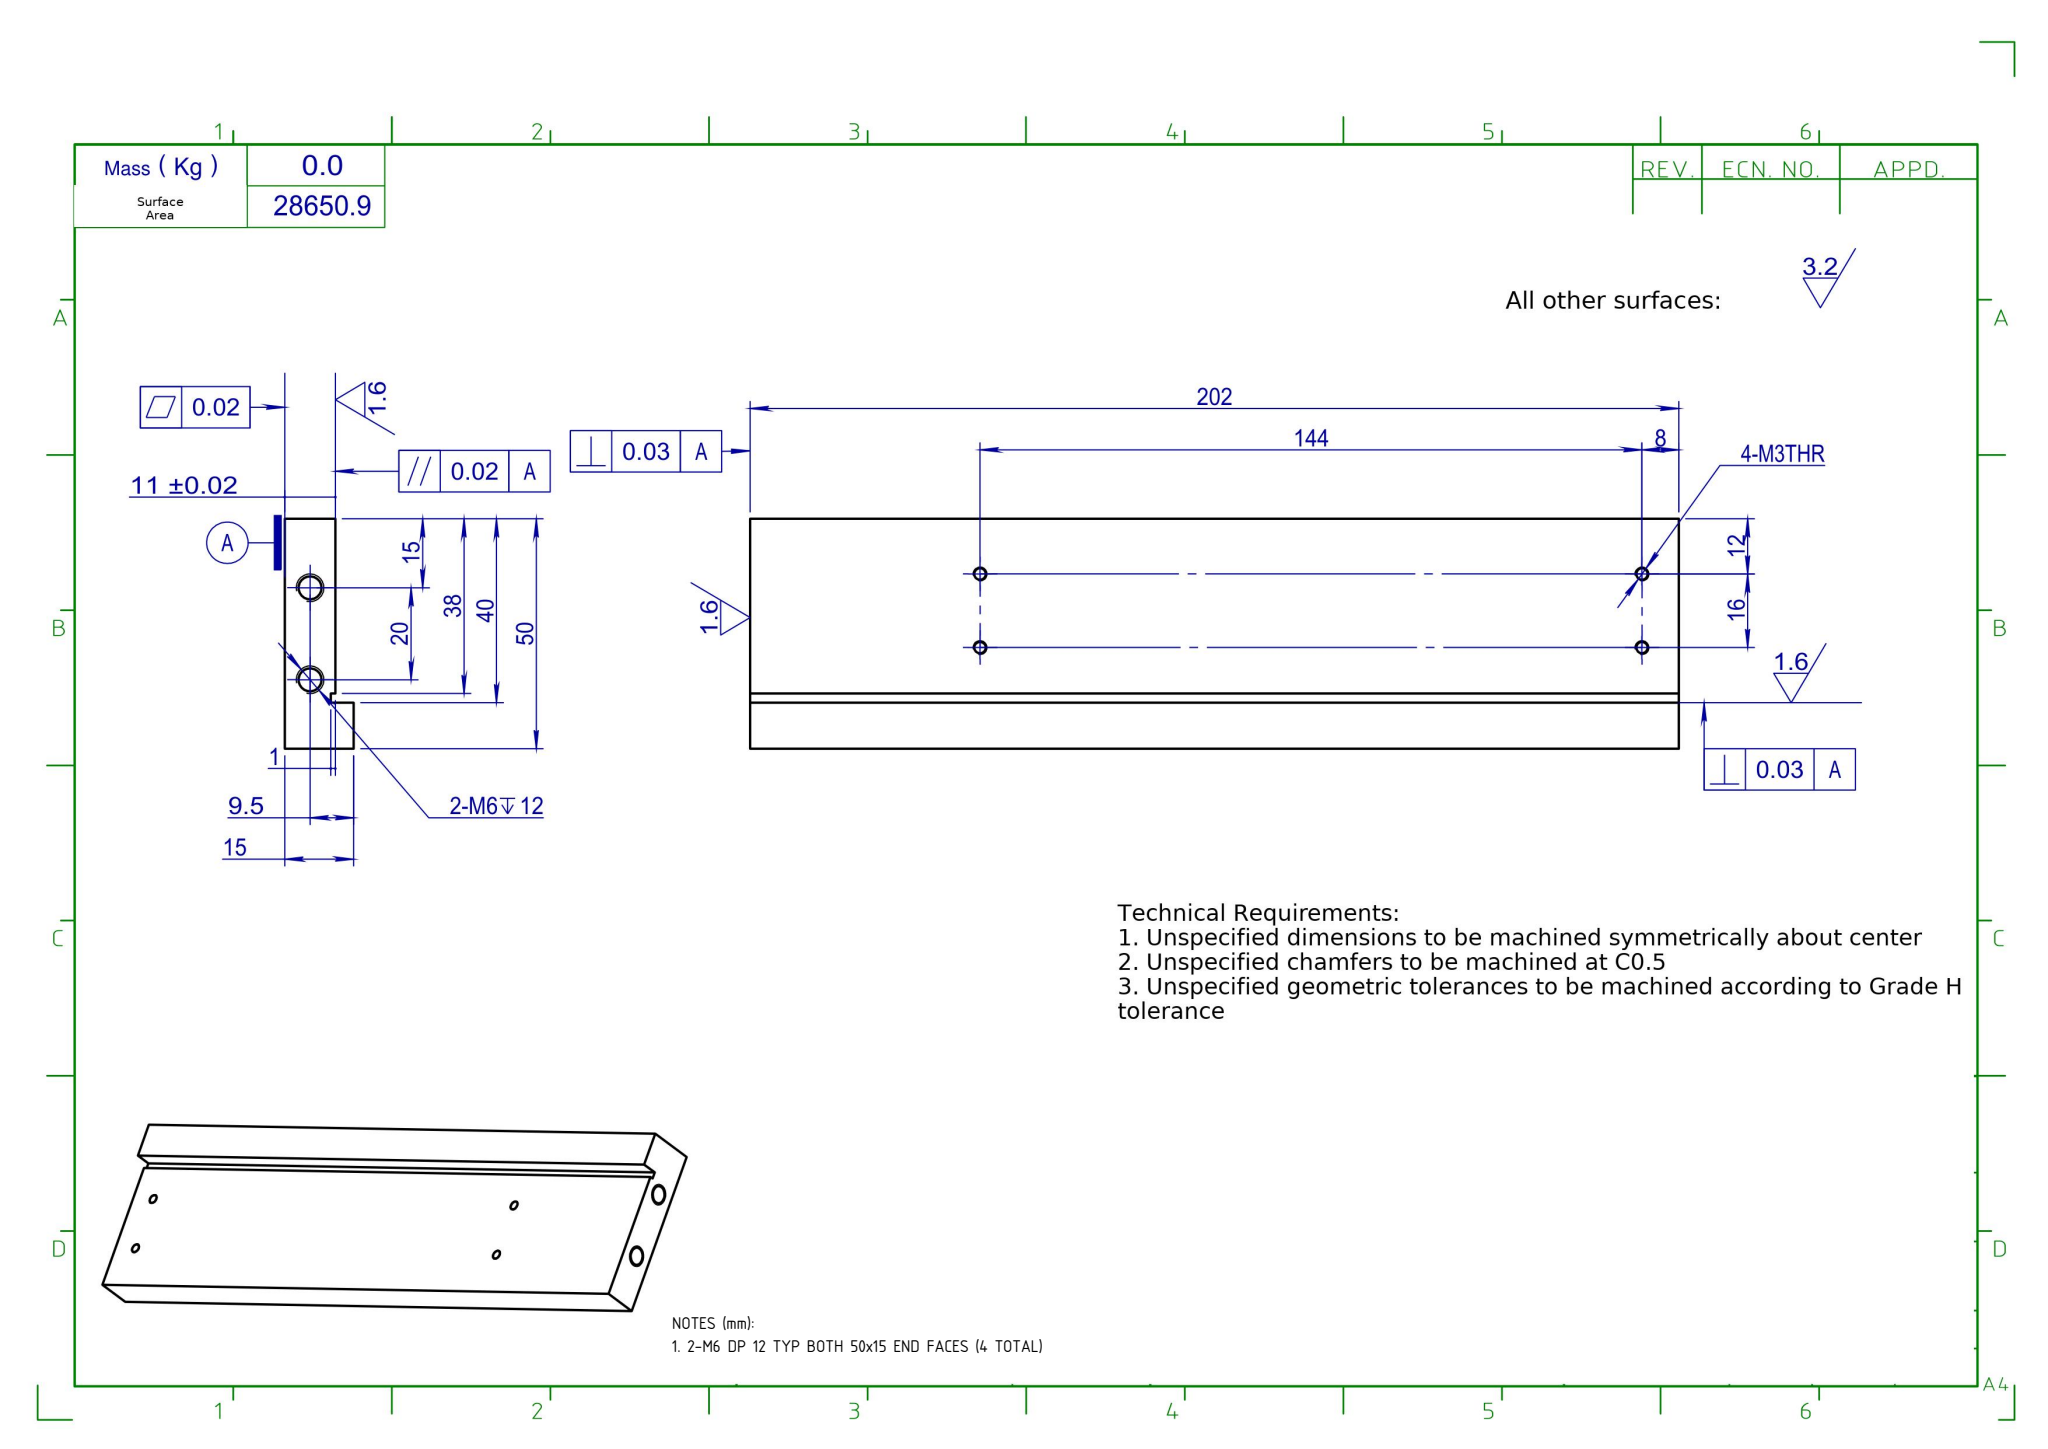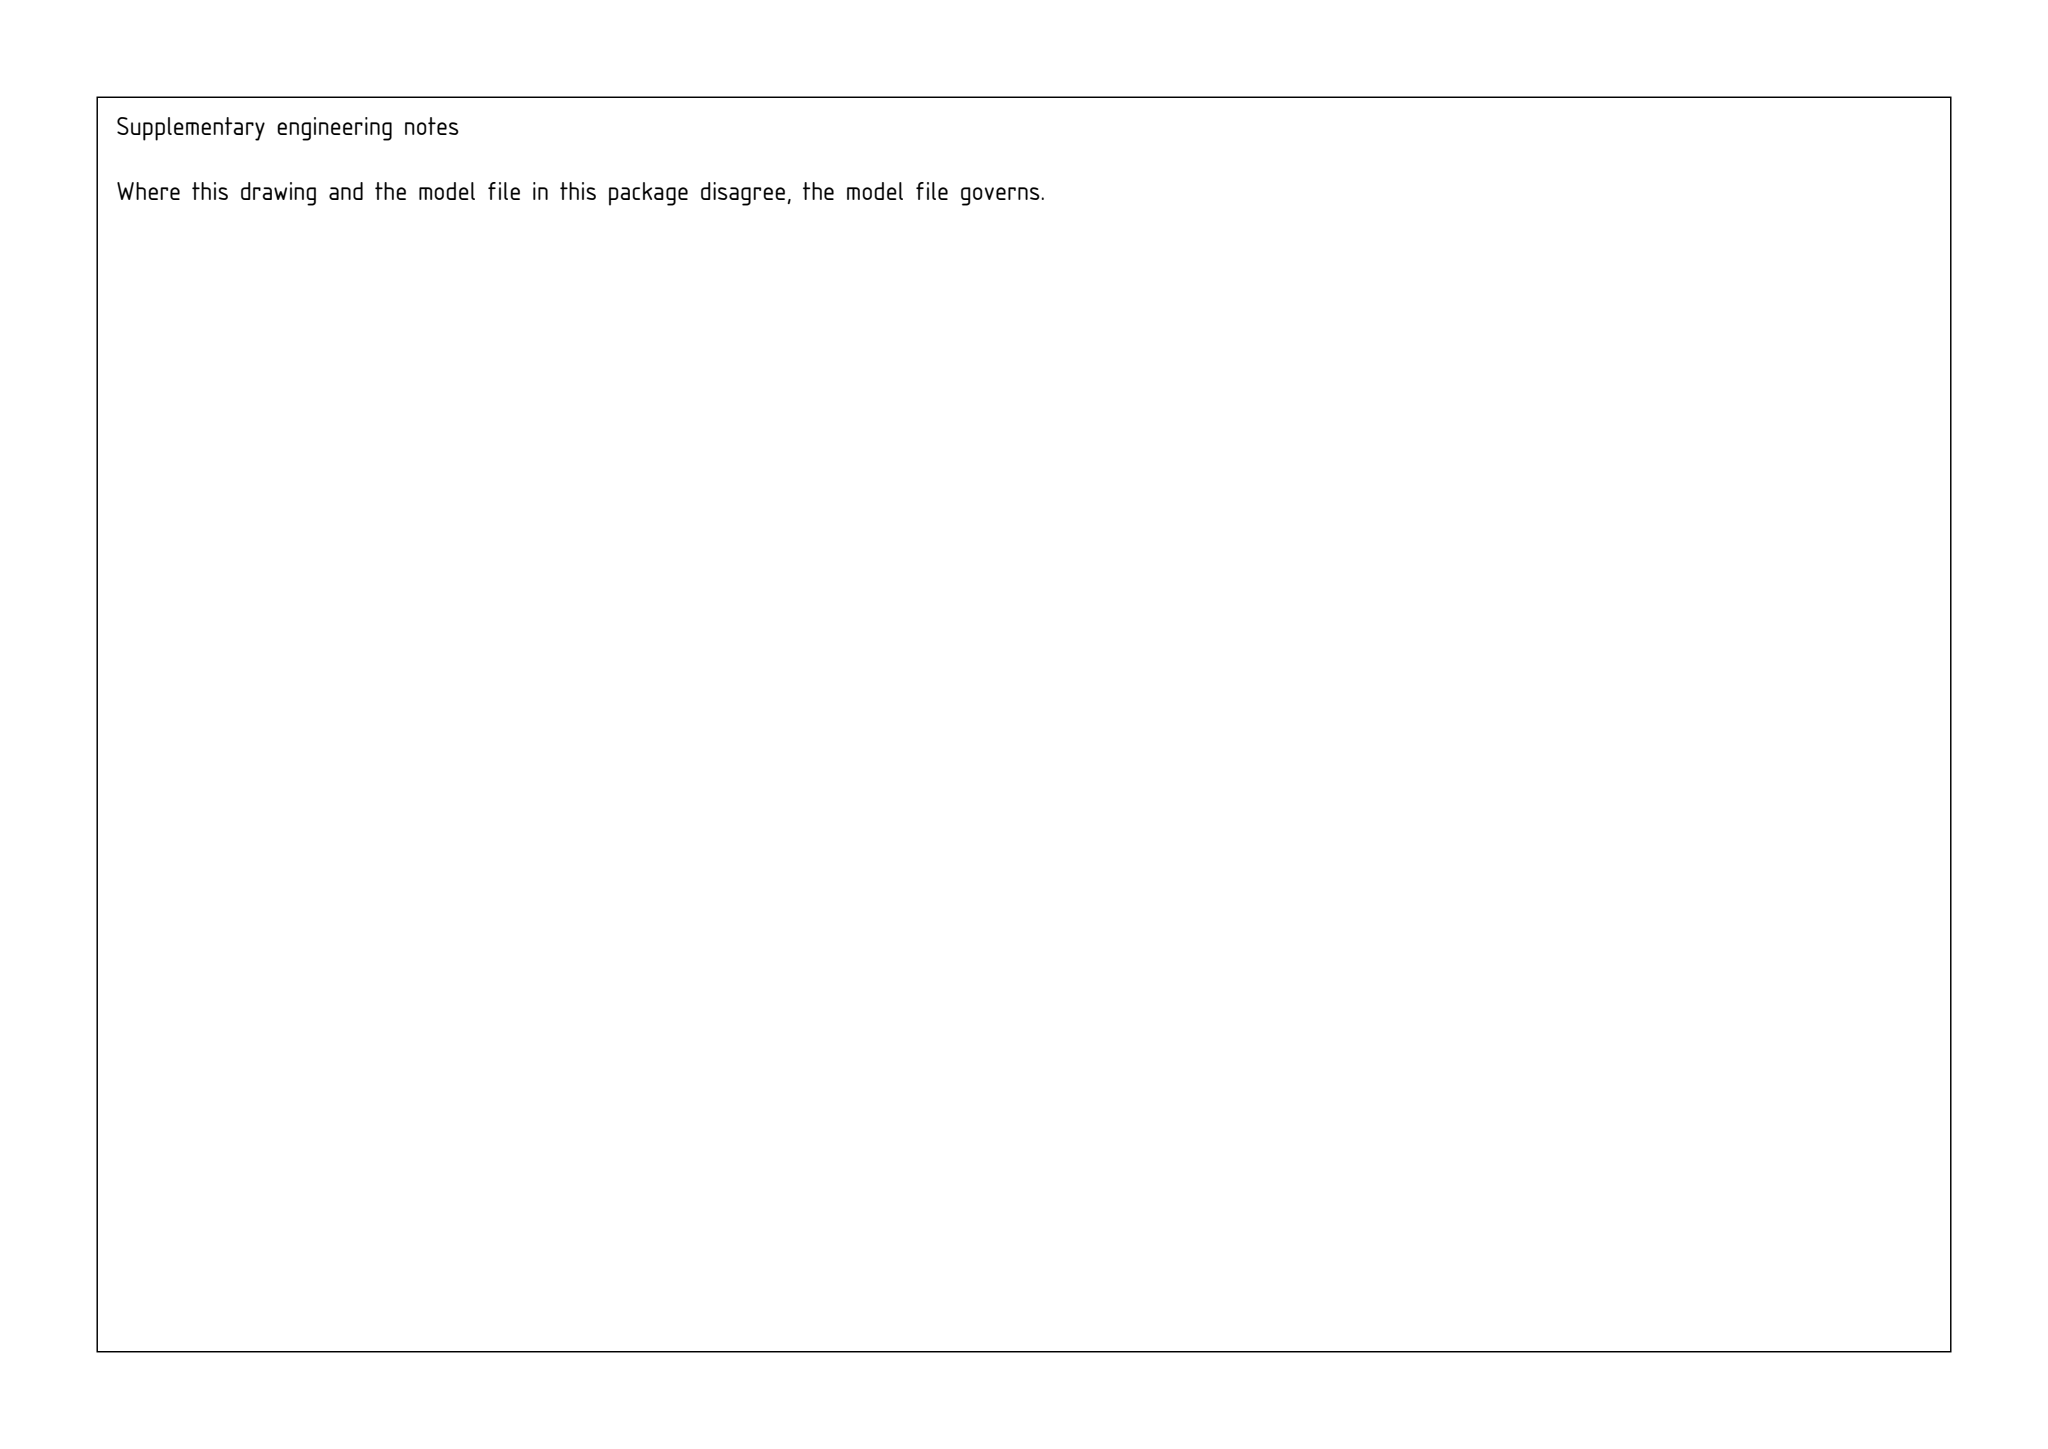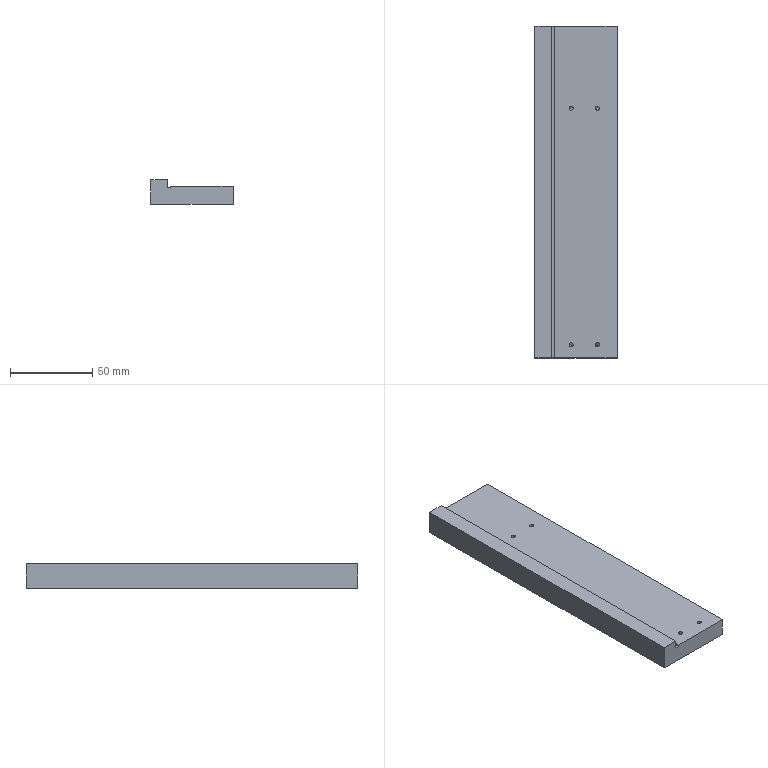Part | SolidWorks | mm | 1 solid | 34 faces | box 50 x 202 x 15 mm | volume 117917 mm3 | cylinder 12 | cone 12 | plane 10 | commonest cylinder face diameters 2.5 x8 5 x4
Drawing notes:
2-M6 DP 12 TYP BOTH 50x15 END FACES (4 TOTAL) | from the solid: Ø5.0 y-axis holes at (x=15,z=5.5) and (x=35,z=5.5), count 2 each, i.e. one pair in each y=0 and y=202 end face; bbox 50x202x15
build123d program:
from build123d import *

# Parameters (mm, degrees)
SKETCH1_W             = 50
SKETCH1_H             = 202
EXTRUDE1_DEPTH        = 15
SKETCH2_W             = 40
SKETCH2_H             = 202
CUT_EXTRUDE1_DEPTH    = 4
SKETCH3_W             = 2
SKETCH3_H             = 202
CUT_EXTRUDE2_DEPTH    = 1
M6_TAPPED_HOLE1_D     = 5
M6_TAPPED_HOLE1_DEPTH = 17
M6_TAPPED_HOLE1_TIP   = 1.502
M3_TAPPED_HOLE1_D     = 2.5
M3_TAPPED_HOLE1_DEPTH = 8.5
M3_TAPPED_HOLE1_TIP   = 0.7511


with BuildPart() as part:
    # Sketch1 → Extrude1 (new body)
    with BuildSketch(Plane.XY):
        Rectangle(SKETCH1_W, SKETCH1_H)
    extrude(amount=EXTRUDE1_DEPTH)

    # Sketch2 → Cut-Extrude1 (cut)
    with BuildSketch(Plane.XY.offset(15)):
        with Locations((5, 0)):
            Rectangle(SKETCH2_W, SKETCH2_H)
    extrude(amount=-CUT_EXTRUDE1_DEPTH, mode=Mode.SUBTRACT)

    # Sketch3 → Cut-Extrude2 (cut)
    with BuildSketch(Plane.XY.offset(11)):
        with Locations((-14, 0)):
            Rectangle(SKETCH3_W, SKETCH3_H)
    extrude(amount=-CUT_EXTRUDE2_DEPTH, mode=Mode.SUBTRACT)

    # M6 Tapped Hole1
    with Locations(Plane(origin=(0, 101, 0), x_dir=(-1, 0, 0), z_dir=(0, 1, 0))):
        with Locations((-10, 5.5), (10, 5.5)):
            Hole(M6_TAPPED_HOLE1_D / 2, depth=M6_TAPPED_HOLE1_DEPTH)
            with Locations((0, 0, -(M6_TAPPED_HOLE1_DEPTH + M6_TAPPED_HOLE1_TIP / 2))):  # 118° drill point
                Cone(0, M6_TAPPED_HOLE1_D / 2, M6_TAPPED_HOLE1_TIP, mode=Mode.SUBTRACT)

    # M3 Tapped Hole1
    with Locations(Plane.XY.offset(11)):
        with Locations((-3, -93), (13, -93), (13, 51), (-3, 51)):
            Hole(M3_TAPPED_HOLE1_D / 2, depth=M3_TAPPED_HOLE1_DEPTH)
            with Locations((0, 0, -(M3_TAPPED_HOLE1_DEPTH + M3_TAPPED_HOLE1_TIP / 2))):  # 118° drill point
                Cone(0, M3_TAPPED_HOLE1_D / 2, M3_TAPPED_HOLE1_TIP, mode=Mode.SUBTRACT)


solid = part.part
STEP:
#1=CARTESIAN_POINT('',(-4.25,-93.,2.5));
#2=VERTEX_POINT('',#1);
#3=CARTESIAN_POINT('',(-1.75,-93.,2.5));
#4=VERTEX_POINT('',#3);
#5=CARTESIAN_POINT('',(-3.,-93.,2.5));
#6=DIRECTION('',(0.,0.,1.));
#7=DIRECTION('',(1.,0.,0.));
#8=AXIS2_PLACEMENT_3D('',#5,#6,#7);
#9=CIRCLE('',#8,1.25);
#10=EDGE_CURVE('',#2,#4,#9,.T.);
#11=ORIENTED_EDGE('',*,*,#10,.F.);
#12=CARTESIAN_POINT('',(-4.25,-93.,11.));
#13=VERTEX_POINT('',#12);
#14=CARTESIAN_POINT('',(-4.25,-93.,11.));
#15=DIRECTION('',(0.,0.,1.));
#16=VECTOR('',#15,1000.);
#17=LINE('',#14,#16);
#18=EDGE_CURVE('',#2,#13,#17,.T.);
#19=ORIENTED_EDGE('',*,*,#18,.T.);
#20=CARTESIAN_POINT('',(-1.75,-93.,11.));
#21=VERTEX_POINT('',#20);
#22=CARTESIAN_POINT('',(-3.,-93.,11.));
#23=DIRECTION('',(0.,0.,1.));
#24=DIRECTION('',(1.,0.,0.));
#25=AXIS2_PLACEMENT_3D('',#22,#23,#24);
#26=CIRCLE('',#25,1.25);
#27=EDGE_CURVE('',#13,#21,#26,.T.);
#28=ORIENTED_EDGE('',*,*,#27,.T.);
#29=CARTESIAN_POINT('',(-1.75,-93.,11.));
#30=DIRECTION('',(0.,0.,1.));
#31=VECTOR('',#30,1000.);
#32=LINE('',#29,#31);
#33=EDGE_CURVE('',#4,#21,#32,.T.);
#34=ORIENTED_EDGE('',*,*,#33,.F.);
#35=EDGE_LOOP('',(#11,#19,#28,#34));
#36=FACE_OUTER_BOUND('',#35,.T.);
#37=CARTESIAN_POINT('',(-3.,-93.,11.));
#38=DIRECTION('',(0.,0.,1.));
#39=DIRECTION('',(1.,0.,0.));
#40=AXIS2_PLACEMENT_3D('',#37,#38,#39);
#41=CYLINDRICAL_SURFACE('',#40,1.25);
#42=ADVANCED_FACE('',(#36),#41,.F.);
#43=CARTESIAN_POINT('',(-3.,-93.,1.749));
#44=VERTEX_POINT('',#43);
#45=CARTESIAN_POINT('',(-1.75,-93.,2.5));
#46=DIRECTION('',(0.8572,0.,0.515));
#47=VECTOR('',#46,1000.);
#48=LINE('',#45,#47);
#49=EDGE_CURVE('',#44,#4,#48,.T.);
#50=ORIENTED_EDGE('',*,*,#49,.F.);
#51=CARTESIAN_POINT('',(-4.25,-93.,2.5));
#52=DIRECTION('',(-0.8572,0.,0.515));
#53=VECTOR('',#52,1000.);
#54=LINE('',#51,#53);
#55=EDGE_CURVE('',#44,#2,#54,.T.);
#56=ORIENTED_EDGE('',*,*,#55,.T.);
#57=ORIENTED_EDGE('',*,*,#10,.T.);
#58=EDGE_LOOP('',(#50,#56,#57));
#59=FACE_OUTER_BOUND('',#58,.T.);
#60=CARTESIAN_POINT('',(-3.,-93.,2.5));
#61=DIRECTION('',(0.,0.,1.));
#62=DIRECTION('',(1.,0.,0.));
#63=AXIS2_PLACEMENT_3D('',#60,#61,#62);
#64=CONICAL_SURFACE('',#63,1.25,1.03);
#65=ADVANCED_FACE('',(#59),#64,.F.);
#66=CARTESIAN_POINT('',(11.75,-93.,2.5));
#67=VERTEX_POINT('',#66);
#68=CARTESIAN_POINT('',(14.25,-93.,2.5));
#69=VERTEX_POINT('',#68);
#70=CARTESIAN_POINT('',(13.,-93.,2.5));
#71=DIRECTION('',(0.,0.,1.));
#72=DIRECTION('',(1.,0.,0.));
#73=AXIS2_PLACEMENT_3D('',#70,#71,#72);
#74=CIRCLE('',#73,1.25);
#75=EDGE_CURVE('',#67,#69,#74,.T.);
#76=ORIENTED_EDGE('',*,*,#75,.F.);
#77=CARTESIAN_POINT('',(11.75,-93.,11.));
#78=VERTEX_POINT('',#77);
#79=CARTESIAN_POINT('',(11.75,-93.,11.));
#80=DIRECTION('',(0.,0.,1.));
#81=VECTOR('',#80,1000.);
#82=LINE('',#79,#81);
#83=EDGE_CURVE('',#67,#78,#82,.T.);
#84=ORIENTED_EDGE('',*,*,#83,.T.);
#85=CARTESIAN_POINT('',(14.25,-93.,11.));
#86=VERTEX_POINT('',#85);
#87=CARTESIAN_POINT('',(13.,-93.,11.));
#88=DIRECTION('',(0.,0.,1.));
#89=DIRECTION('',(1.,0.,0.));
#90=AXIS2_PLACEMENT_3D('',#87,#88,#89);
#91=CIRCLE('',#90,1.25);
#92=EDGE_CURVE('',#78,#86,#91,.T.);
#93=ORIENTED_EDGE('',*,*,#92,.T.);
#94=CARTESIAN_POINT('',(14.25,-93.,11.));
#95=DIRECTION('',(0.,0.,1.));
#96=VECTOR('',#95,1000.);
#97=LINE('',#94,#96);
#98=EDGE_CURVE('',#69,#86,#97,.T.);
#99=ORIENTED_EDGE('',*,*,#98,.F.);
#100=EDGE_LOOP('',(#76,#84,#93,#99));
#101=FACE_OUTER_BOUND('',#100,.T.);
#102=CARTESIAN_POINT('',(13.,-93.,11.));
#103=DIRECTION('',(0.,0.,1.));
#104=DIRECTION('',(1.,0.,0.));
#105=AXIS2_PLACEMENT_3D('',#102,#103,#104);
#106=CYLINDRICAL_SURFACE('',#105,1.25);
#107=ADVANCED_FACE('',(#101),#106,.F.);
#108=CARTESIAN_POINT('',(13.,-93.,1.749));
#109=VERTEX_POINT('',#108);
#110=CARTESIAN_POINT('',(14.25,-93.,2.5));
#111=DIRECTION('',(0.8572,0.,0.515));
#112=VECTOR('',#111,1000.);
#113=LINE('',#110,#112);
#114=EDGE_CURVE('',#109,#69,#113,.T.);
#115=ORIENTED_EDGE('',*,*,#114,.F.);
#116=CARTESIAN_POINT('',(11.75,-93.,2.5));
#117=DIRECTION('',(-0.8572,0.,0.515));
#118=VECTOR('',#117,1000.);
#119=LINE('',#116,#118);
#120=EDGE_CURVE('',#109,#67,#119,.T.);
#121=ORIENTED_EDGE('',*,*,#120,.T.);
#122=ORIENTED_EDGE('',*,*,#75,.T.);
#123=EDGE_LOOP('',(#115,#121,#122));
#124=FACE_OUTER_BOUND('',#123,.T.);
#125=CARTESIAN_POINT('',(13.,-93.,2.5));
#126=DIRECTION('',(0.,0.,1.));
#127=DIRECTION('',(1.,0.,0.));
#128=AXIS2_PLACEMENT_3D('',#125,#126,#127);
#129=CONICAL_SURFACE('',#128,1.25,1.03);
#130=ADVANCED_FACE('',(#124),#129,.F.);
#131=CARTESIAN_POINT('',(11.75,51.,2.5));
#132=VERTEX_POINT('',#131);
#133=CARTESIAN_POINT('',(14.25,51.,2.5));
#134=VERTEX_POINT('',#133);
#135=CARTESIAN_POINT('',(13.,51.,2.5));
#136=DIRECTION('',(0.,0.,1.));
#137=DIRECTION('',(1.,0.,0.));
#138=AXIS2_PLACEMENT_3D('',#135,#136,#137);
#139=CIRCLE('',#138,1.25);
#140=EDGE_CURVE('',#132,#134,#139,.T.);
#141=ORIENTED_EDGE('',*,*,#140,.F.);
#142=CARTESIAN_POINT('',(11.75,51.,11.));
#143=VERTEX_POINT('',#142);
#144=CARTESIAN_POINT('',(11.75,51.,11.));
#145=DIRECTION('',(0.,0.,1.));
#146=VECTOR('',#145,1000.);
#147=LINE('',#144,#146);
#148=EDGE_CURVE('',#132,#143,#147,.T.);
#149=ORIENTED_EDGE('',*,*,#148,.T.);
#150=CARTESIAN_POINT('',(14.25,51.,11.));
#151=VERTEX_POINT('',#150);
#152=CARTESIAN_POINT('',(13.,51.,11.));
#153=DIRECTION('',(0.,0.,1.));
#154=DIRECTION('',(1.,0.,0.));
#155=AXIS2_PLACEMENT_3D('',#152,#153,#154);
#156=CIRCLE('',#155,1.25);
#157=EDGE_CURVE('',#143,#151,#156,.T.);
#158=ORIENTED_EDGE('',*,*,#157,.T.);
#159=CARTESIAN_POINT('',(14.25,51.,11.));
#160=DIRECTION('',(0.,0.,1.));
#161=VECTOR('',#160,1000.);
#162=LINE('',#159,#161);
#163=EDGE_CURVE('',#134,#151,#162,.T.);
#164=ORIENTED_EDGE('',*,*,#163,.F.);
#165=EDGE_LOOP('',(#141,#149,#158,#164));
#166=FACE_OUTER_BOUND('',#165,.T.);
#167=CARTESIAN_POINT('',(13.,51.,11.));
#168=DIRECTION('',(0.,0.,1.));
#169=DIRECTION('',(1.,0.,0.));
#170=AXIS2_PLACEMENT_3D('',#167,#168,#169);
#171=CYLINDRICAL_SURFACE('',#170,1.25);
#172=ADVANCED_FACE('',(#166),#171,.F.);
#173=CARTESIAN_POINT('',(13.,51.,1.749));
#174=VERTEX_POINT('',#173);
#175=CARTESIAN_POINT('',(14.25,51.,2.5));
#176=DIRECTION('',(0.8572,0.,0.515));
#177=VECTOR('',#176,1000.);
#178=LINE('',#175,#177);
#179=EDGE_CURVE('',#174,#134,#178,.T.);
#180=ORIENTED_EDGE('',*,*,#179,.F.);
#181=CARTESIAN_POINT('',(11.75,51.,2.5));
#182=DIRECTION('',(-0.8572,0.,0.515));
#183=VECTOR('',#182,1000.);
#184=LINE('',#181,#183);
#185=EDGE_CURVE('',#174,#132,#184,.T.);
#186=ORIENTED_EDGE('',*,*,#185,.T.);
#187=ORIENTED_EDGE('',*,*,#140,.T.);
#188=EDGE_LOOP('',(#180,#186,#187));
#189=FACE_OUTER_BOUND('',#188,.T.);
#190=CARTESIAN_POINT('',(13.,51.,2.5));
#191=DIRECTION('',(0.,0.,1.));
#192=DIRECTION('',(1.,0.,0.));
#193=AXIS2_PLACEMENT_3D('',#190,#191,#192);
#194=CONICAL_SURFACE('',#193,1.25,1.03);
#195=ADVANCED_FACE('',(#189),#194,.F.);
#196=CARTESIAN_POINT('',(-4.25,51.,2.5));
#197=VERTEX_POINT('',#196);
#198=CARTESIAN_POINT('',(-1.75,51.,2.5));
#199=VERTEX_POINT('',#198);
#200=CARTESIAN_POINT('',(-3.,51.,2.5));
#201=DIRECTION('',(0.,0.,1.));
#202=DIRECTION('',(1.,0.,0.));
#203=AXIS2_PLACEMENT_3D('',#200,#201,#202);
#204=CIRCLE('',#203,1.25);
#205=EDGE_CURVE('',#197,#199,#204,.T.);
#206=ORIENTED_EDGE('',*,*,#205,.F.);
#207=CARTESIAN_POINT('',(-4.25,51.,11.));
#208=VERTEX_POINT('',#207);
#209=CARTESIAN_POINT('',(-4.25,51.,11.));
#210=DIRECTION('',(0.,0.,1.));
#211=VECTOR('',#210,1000.);
#212=LINE('',#209,#211);
#213=EDGE_CURVE('',#197,#208,#212,.T.);
#214=ORIENTED_EDGE('',*,*,#213,.T.);
#215=CARTESIAN_POINT('',(-1.75,51.,11.));
#216=VERTEX_POINT('',#215);
#217=CARTESIAN_POINT('',(-3.,51.,11.));
#218=DIRECTION('',(0.,0.,1.));
#219=DIRECTION('',(1.,0.,0.));
#220=AXIS2_PLACEMENT_3D('',#217,#218,#219);
#221=CIRCLE('',#220,1.25);
#222=EDGE_CURVE('',#208,#216,#221,.T.);
#223=ORIENTED_EDGE('',*,*,#222,.T.);
#224=CARTESIAN_POINT('',(-1.75,51.,11.));
#225=DIRECTION('',(0.,0.,1.));
#226=VECTOR('',#225,1000.);
#227=LINE('',#224,#226);
#228=EDGE_CURVE('',#199,#216,#227,.T.);
#229=ORIENTED_EDGE('',*,*,#228,.F.);
#230=EDGE_LOOP('',(#206,#214,#223,#229));
#231=FACE_OUTER_BOUND('',#230,.T.);
#232=CARTESIAN_POINT('',(-3.,51.,11.));
#233=DIRECTION('',(0.,0.,1.));
#234=DIRECTION('',(1.,0.,0.));
#235=AXIS2_PLACEMENT_3D('',#232,#233,#234);
#236=CYLINDRICAL_SURFACE('',#235,1.25);
#237=ADVANCED_FACE('',(#231),#236,.F.);
#238=CARTESIAN_POINT('',(-3.,51.,1.749));
#239=VERTEX_POINT('',#238);
#240=CARTESIAN_POINT('',(-1.75,51.,2.5));
#241=DIRECTION('',(0.8572,0.,0.515));
#242=VECTOR('',#241,1000.);
#243=LINE('',#240,#242);
#244=EDGE_CURVE('',#239,#199,#243,.T.);
#245=ORIENTED_EDGE('',*,*,#244,.F.);
#246=CARTESIAN_POINT('',(-4.25,51.,2.5));
#247=DIRECTION('',(-0.8572,0.,0.515));
#248=VECTOR('',#247,1000.);
#249=LINE('',#246,#248);
#250=EDGE_CURVE('',#239,#197,#249,.T.);
#251=ORIENTED_EDGE('',*,*,#250,.T.);
#252=ORIENTED_EDGE('',*,*,#205,.T.);
#253=EDGE_LOOP('',(#245,#251,#252));
#254=FACE_OUTER_BOUND('',#253,.T.);
#255=CARTESIAN_POINT('',(-3.,51.,2.5));
#256=DIRECTION('',(0.,0.,1.));
#257=DIRECTION('',(1.,0.,0.));
#258=AXIS2_PLACEMENT_3D('',#255,#256,#257);
#259=CONICAL_SURFACE('',#258,1.25,1.03);
#260=ADVANCED_FACE('',(#254),#259,.F.);
#261=CARTESIAN_POINT('',(10.,82.498,5.5));
#262=VERTEX_POINT('',#261);
#263=CARTESIAN_POINT('',(10.,84.,8.));
#264=VERTEX_POINT('',#263);
#265=CARTESIAN_POINT('',(10.,84.,8.));
#266=DIRECTION('',(0.,0.515,0.8572));
#267=VECTOR('',#266,1000.);
#268=LINE('',#265,#267);
#269=EDGE_CURVE('',#262,#264,#268,.T.);
#270=ORIENTED_EDGE('',*,*,#269,.F.);
#271=CARTESIAN_POINT('',(10.,84.,3.));
#272=VERTEX_POINT('',#271);
#273=CARTESIAN_POINT('',(10.,84.,3.));
#274=DIRECTION('',(0.,0.515,-0.8572));
#275=VECTOR('',#274,1000.);
#276=LINE('',#273,#275);
#277=EDGE_CURVE('',#262,#272,#276,.T.);
#278=ORIENTED_EDGE('',*,*,#277,.T.);
#279=CARTESIAN_POINT('',(10.,84.,5.5));
#280=DIRECTION('',(0.,1.,0.));
#281=DIRECTION('',(0.,0.,1.));
#282=AXIS2_PLACEMENT_3D('',#279,#280,#281);
#283=CIRCLE('',#282,2.5);
#284=EDGE_CURVE('',#272,#264,#283,.T.);
#285=ORIENTED_EDGE('',*,*,#284,.T.);
#286=EDGE_LOOP('',(#270,#278,#285));
#287=FACE_OUTER_BOUND('',#286,.T.);
#288=CARTESIAN_POINT('',(10.,84.,5.5));
#289=DIRECTION('',(0.,1.,0.));
#290=DIRECTION('',(0.,0.,1.));
#291=AXIS2_PLACEMENT_3D('',#288,#289,#290);
#292=CONICAL_SURFACE('',#291,2.5,1.03);
#293=ADVANCED_FACE('',(#287),#292,.F.);
#294=ORIENTED_EDGE('',*,*,#284,.F.);
#295=CARTESIAN_POINT('',(10.,101.,3.));
#296=VERTEX_POINT('',#295);
#297=CARTESIAN_POINT('',(10.,101.,3.));
#298=DIRECTION('',(0.,1.,0.));
#299=VECTOR('',#298,1000.);
#300=LINE('',#297,#299);
#301=EDGE_CURVE('',#272,#296,#300,.T.);
#302=ORIENTED_EDGE('',*,*,#301,.T.);
#303=CARTESIAN_POINT('',(10.,101.,8.));
#304=VERTEX_POINT('',#303);
#305=CARTESIAN_POINT('',(10.,101.,5.5));
#306=DIRECTION('',(0.,1.,0.));
#307=DIRECTION('',(0.,0.,1.));
#308=AXIS2_PLACEMENT_3D('',#305,#306,#307);
#309=CIRCLE('',#308,2.5);
#310=EDGE_CURVE('',#296,#304,#309,.T.);
#311=ORIENTED_EDGE('',*,*,#310,.T.);
#312=CARTESIAN_POINT('',(10.,101.,8.));
#313=DIRECTION('',(0.,1.,0.));
#314=VECTOR('',#313,1000.);
#315=LINE('',#312,#314);
#316=EDGE_CURVE('',#264,#304,#315,.T.);
#317=ORIENTED_EDGE('',*,*,#316,.F.);
#318=EDGE_LOOP('',(#294,#302,#311,#317));
#319=FACE_OUTER_BOUND('',#318,.T.);
#320=CARTESIAN_POINT('',(10.,101.,5.5));
#321=DIRECTION('',(0.,1.,0.));
#322=DIRECTION('',(0.,0.,1.));
#323=AXIS2_PLACEMENT_3D('',#320,#321,#322);
#324=CYLINDRICAL_SURFACE('',#323,2.5);
#325=ADVANCED_FACE('',(#319),#324,.F.);
#326=CARTESIAN_POINT('',(-10.,82.498,5.5));
#327=VERTEX_POINT('',#326);
#328=CARTESIAN_POINT('',(-10.,84.,8.));
#329=VERTEX_POINT('',#328);
#330=CARTESIAN_POINT('',(-10.,84.,8.));
#331=DIRECTION('',(0.,0.515,0.8572));
#332=VECTOR('',#331,1000.);
#333=LINE('',#330,#332);
#334=EDGE_CURVE('',#327,#329,#333,.T.);
#335=ORIENTED_EDGE('',*,*,#334,.F.);
#336=CARTESIAN_POINT('',(-10.,84.,3.));
#337=VERTEX_POINT('',#336);
#338=CARTESIAN_POINT('',(-10.,84.,3.));
#339=DIRECTION('',(0.,0.515,-0.8572));
#340=VECTOR('',#339,1000.);
#341=LINE('',#338,#340);
#342=EDGE_CURVE('',#327,#337,#341,.T.);
#343=ORIENTED_EDGE('',*,*,#342,.T.);
#344=CARTESIAN_POINT('',(-10.,84.,5.5));
#345=DIRECTION('',(0.,1.,0.));
#346=DIRECTION('',(0.,0.,1.));
#347=AXIS2_PLACEMENT_3D('',#344,#345,#346);
#348=CIRCLE('',#347,2.5);
#349=EDGE_CURVE('',#337,#329,#348,.T.);
#350=ORIENTED_EDGE('',*,*,#349,.T.);
#351=EDGE_LOOP('',(#335,#343,#350));
#352=FACE_OUTER_BOUND('',#351,.T.);
#353=CARTESIAN_POINT('',(-10.,84.,5.5));
#354=DIRECTION('',(0.,1.,0.));
#355=DIRECTION('',(0.,0.,1.));
#356=AXIS2_PLACEMENT_3D('',#353,#354,#355);
#357=CONICAL_SURFACE('',#356,2.5,1.03);
#358=ADVANCED_FACE('',(#352),#357,.F.);
#359=ORIENTED_EDGE('',*,*,#349,.F.);
#360=CARTESIAN_POINT('',(-10.,101.,3.));
#361=VERTEX_POINT('',#360);
#362=CARTESIAN_POINT('',(-10.,101.,3.));
#363=DIRECTION('',(0.,1.,0.));
#364=VECTOR('',#363,1000.);
#365=LINE('',#362,#364);
#366=EDGE_CURVE('',#337,#361,#365,.T.);
#367=ORIENTED_EDGE('',*,*,#366,.T.);
#368=CARTESIAN_POINT('',(-10.,101.,8.));
#369=VERTEX_POINT('',#368);
#370=CARTESIAN_POINT('',(-10.,101.,5.5));
#371=DIRECTION('',(0.,1.,0.));
#372=DIRECTION('',(0.,0.,1.));
#373=AXIS2_PLACEMENT_3D('',#370,#371,#372);
#374=CIRCLE('',#373,2.5);
#375=EDGE_CURVE('',#361,#369,#374,.T.);
#376=ORIENTED_EDGE('',*,*,#375,.T.);
#377=CARTESIAN_POINT('',(-10.,101.,8.));
#378=DIRECTION('',(0.,1.,0.));
#379=VECTOR('',#378,1000.);
#380=LINE('',#377,#379);
#381=EDGE_CURVE('',#329,#369,#380,.T.);
#382=ORIENTED_EDGE('',*,*,#381,.F.);
#383=EDGE_LOOP('',(#359,#367,#376,#382));
#384=FACE_OUTER_BOUND('',#383,.T.);
#385=CARTESIAN_POINT('',(-10.,101.,5.5));
#386=DIRECTION('',(0.,1.,0.));
#387=DIRECTION('',(0.,0.,1.));
#388=AXIS2_PLACEMENT_3D('',#385,#386,#387);
#389=CYLINDRICAL_SURFACE('',#388,2.5);
#390=ADVANCED_FACE('',(#384),#389,.F.);
#391=CARTESIAN_POINT('',(25.,-101.,11.));
#392=VERTEX_POINT('',#391);
#393=CARTESIAN_POINT('',(25.,101.,11.));
#394=VERTEX_POINT('',#393);
#395=CARTESIAN_POINT('',(25.,101.,11.));
#396=DIRECTION('',(-0.,1.,0.));
#397=VECTOR('',#396,1000.);
#398=LINE('',#395,#397);
#399=EDGE_CURVE('',#392,#394,#398,.T.);
#400=ORIENTED_EDGE('',*,*,#399,.F.);
#401=CARTESIAN_POINT('',(25.,-101.,0.));
#402=VERTEX_POINT('',#401);
#403=CARTESIAN_POINT('',(25.,-101.,15.));
#404=DIRECTION('',(0.,0.,-1.));
#405=VECTOR('',#404,1000.);
#406=LINE('',#403,#405);
#407=EDGE_CURVE('',#392,#402,#406,.T.);
#408=ORIENTED_EDGE('',*,*,#407,.T.);
#409=CARTESIAN_POINT('',(25.,101.,0.));
#410=VERTEX_POINT('',#409);
#411=CARTESIAN_POINT('',(25.,101.,0.));
#412=DIRECTION('',(-0.,1.,0.));
#413=VECTOR('',#412,1000.);
#414=LINE('',#411,#413);
#415=EDGE_CURVE('',#402,#410,#414,.T.);
#416=ORIENTED_EDGE('',*,*,#415,.T.);
#417=CARTESIAN_POINT('',(25.,101.,15.));
#418=DIRECTION('',(0.,0.,-1.));
#419=VECTOR('',#418,1000.);
#420=LINE('',#417,#419);
#421=EDGE_CURVE('',#394,#410,#420,.T.);
#422=ORIENTED_EDGE('',*,*,#421,.F.);
#423=EDGE_LOOP('',(#400,#408,#416,#422));
#424=FACE_OUTER_BOUND('',#423,.T.);
#425=CARTESIAN_POINT('',(25.,101.,15.));
#426=DIRECTION('',(-1.,-0.,0.));
#427=DIRECTION('',(0.,-1.,0.));
#428=AXIS2_PLACEMENT_3D('',#425,#426,#427);
#429=PLANE('',#428);
#430=ADVANCED_FACE('',(#424),#429,.F.);
#431=CARTESIAN_POINT('',(-25.,101.,0.));
#432=VERTEX_POINT('',#431);
#433=CARTESIAN_POINT('',(-25.,-101.,0.));
#434=VERTEX_POINT('',#433);
#435=CARTESIAN_POINT('',(-25.,101.,0.));
#436=DIRECTION('',(0.,-1.,0.));
#437=VECTOR('',#436,1000.);
#438=LINE('',#435,#437);
#439=EDGE_CURVE('',#432,#434,#438,.T.);
#440=ORIENTED_EDGE('',*,*,#439,.T.);
#441=CARTESIAN_POINT('',(-25.,-101.,15.));
#442=VERTEX_POINT('',#441);
#443=CARTESIAN_POINT('',(-25.,-101.,15.));
#444=DIRECTION('',(0.,0.,-1.));
#445=VECTOR('',#444,1000.);
#446=LINE('',#443,#445);
#447=EDGE_CURVE('',#442,#434,#446,.T.);
#448=ORIENTED_EDGE('',*,*,#447,.F.);
#449=CARTESIAN_POINT('',(-25.,101.,15.));
#450=VERTEX_POINT('',#449);
#451=CARTESIAN_POINT('',(-25.,101.,15.));
#452=DIRECTION('',(0.,-1.,0.));
#453=VECTOR('',#452,1000.);
#454=LINE('',#451,#453);
#455=EDGE_CURVE('',#450,#442,#454,.T.);
#456=ORIENTED_EDGE('',*,*,#455,.F.);
#457=CARTESIAN_POINT('',(-25.,101.,15.));
#458=DIRECTION('',(0.,0.,-1.));
#459=VECTOR('',#458,1000.);
#460=LINE('',#457,#459);
#461=EDGE_CURVE('',#450,#432,#460,.T.);
#462=ORIENTED_EDGE('',*,*,#461,.T.);
#463=EDGE_LOOP('',(#440,#448,#456,#462));
#464=FACE_OUTER_BOUND('',#463,.T.);
#465=CARTESIAN_POINT('',(-25.,101.,15.));
#466=DIRECTION('',(1.,0.,0.));
#467=DIRECTION('',(-0.,1.,0.));
#468=AXIS2_PLACEMENT_3D('',#465,#466,#467);
#469=PLANE('',#468);
#470=ADVANCED_FACE('',(#464),#469,.F.);
#471=CARTESIAN_POINT('',(-15.,-101.,10.));
#472=VERTEX_POINT('',#471);
#473=CARTESIAN_POINT('',(-13.,-101.,10.));
#474=VERTEX_POINT('',#473);
#475=CARTESIAN_POINT('',(-15.,-101.,10.));
#476=DIRECTION('',(1.,0.,0.));
#477=VECTOR('',#476,1000.);
#478=LINE('',#475,#477);
#479=EDGE_CURVE('',#472,#474,#478,.T.);
#480=ORIENTED_EDGE('',*,*,#479,.F.);
#481=CARTESIAN_POINT('',(-15.,-101.,15.));
#482=VERTEX_POINT('',#481);
#483=CARTESIAN_POINT('',(-15.,-101.,11.));
#484=DIRECTION('',(0.,0.,1.));
#485=VECTOR('',#484,1000.);
#486=LINE('',#483,#485);
#487=EDGE_CURVE('',#472,#482,#486,.T.);
#488=ORIENTED_EDGE('',*,*,#487,.T.);
#489=CARTESIAN_POINT('',(-25.,-101.,15.));
#490=DIRECTION('',(1.,0.,0.));
#491=VECTOR('',#490,1000.);
#492=LINE('',#489,#491);
#493=EDGE_CURVE('',#442,#482,#492,.T.);
#494=ORIENTED_EDGE('',*,*,#493,.F.);
#495=ORIENTED_EDGE('',*,*,#447,.T.);
#496=CARTESIAN_POINT('',(-25.,-101.,0.));
#497=DIRECTION('',(1.,0.,0.));
#498=VECTOR('',#497,1000.);
#499=LINE('',#496,#498);
#500=EDGE_CURVE('',#434,#402,#499,.T.);
#501=ORIENTED_EDGE('',*,*,#500,.T.);
#502=ORIENTED_EDGE('',*,*,#407,.F.);
#503=CARTESIAN_POINT('',(-13.,-101.,11.));
#504=VERTEX_POINT('',#503);
#505=CARTESIAN_POINT('',(-15.,-101.,11.));
#506=DIRECTION('',(1.,0.,0.));
#507=VECTOR('',#506,1000.);
#508=LINE('',#505,#507);
#509=EDGE_CURVE('',#504,#392,#508,.T.);
#510=ORIENTED_EDGE('',*,*,#509,.F.);
#511=CARTESIAN_POINT('',(-13.,-101.,10.));
#512=DIRECTION('',(0.,0.,1.));
#513=VECTOR('',#512,1000.);
#514=LINE('',#511,#513);
#515=EDGE_CURVE('',#474,#504,#514,.T.);
#516=ORIENTED_EDGE('',*,*,#515,.F.);
#517=EDGE_LOOP('',(#480,#488,#494,#495,#501,#502,#510,#516));
#518=FACE_OUTER_BOUND('',#517,.T.);
#519=CARTESIAN_POINT('',(-25.,-101.,15.));
#520=DIRECTION('',(0.,1.,0.));
#521=DIRECTION('',(0.,0.,1.));
#522=AXIS2_PLACEMENT_3D('',#519,#520,#521);
#523=PLANE('',#522);
#524=ADVANCED_FACE('',(#518),#523,.F.);
#525=CARTESIAN_POINT('',(10.,101.,5.5));
#526=DIRECTION('',(0.,1.,0.));
#527=DIRECTION('',(0.,0.,1.));
#528=AXIS2_PLACEMENT_3D('',#525,#526,#527);
#529=CIRCLE('',#528,2.5);
#530=EDGE_CURVE('',#304,#296,#529,.T.);
#531=ORIENTED_EDGE('',*,*,#530,.F.);
#532=ORIENTED_EDGE('',*,*,#310,.F.);
#533=EDGE_LOOP('',(#531,#532));
#534=FACE_BOUND('',#533,.T.);
#535=CARTESIAN_POINT('',(-10.,101.,5.5));
#536=DIRECTION('',(0.,1.,0.));
#537=DIRECTION('',(0.,0.,1.));
#538=AXIS2_PLACEMENT_3D('',#535,#536,#537);
#539=CIRCLE('',#538,2.5);
#540=EDGE_CURVE('',#369,#361,#539,.T.);
#541=ORIENTED_EDGE('',*,*,#540,.F.);
#542=ORIENTED_EDGE('',*,*,#375,.F.);
#543=EDGE_LOOP('',(#541,#542));
#544=FACE_BOUND('',#543,.T.);
#545=CARTESIAN_POINT('',(-15.,101.,10.));
#546=VERTEX_POINT('',#545);
#547=CARTESIAN_POINT('',(-15.,101.,15.));
#548=VERTEX_POINT('',#547);
#549=CARTESIAN_POINT('',(-15.,101.,11.));
#550=DIRECTION('',(0.,0.,1.));
#551=VECTOR('',#550,1000.);
#552=LINE('',#549,#551);
#553=EDGE_CURVE('',#546,#548,#552,.T.);
#554=ORIENTED_EDGE('',*,*,#553,.F.);
#555=CARTESIAN_POINT('',(-13.,101.,10.));
#556=VERTEX_POINT('',#555);
#557=CARTESIAN_POINT('',(-15.,101.,10.));
#558=DIRECTION('',(-1.,0.,0.));
#559=VECTOR('',#558,1000.);
#560=LINE('',#557,#559);
#561=EDGE_CURVE('',#556,#546,#560,.T.);
#562=ORIENTED_EDGE('',*,*,#561,.F.);
#563=CARTESIAN_POINT('',(-13.,101.,11.));
#564=VERTEX_POINT('',#563);
#565=CARTESIAN_POINT('',(-13.,101.,10.));
#566=DIRECTION('',(0.,0.,1.));
#567=VECTOR('',#566,1000.);
#568=LINE('',#565,#567);
#569=EDGE_CURVE('',#556,#564,#568,.T.);
#570=ORIENTED_EDGE('',*,*,#569,.T.);
#571=CARTESIAN_POINT('',(-15.,101.,11.));
#572=DIRECTION('',(-1.,0.,0.));
#573=VECTOR('',#572,1000.);
#574=LINE('',#571,#573);
#575=EDGE_CURVE('',#394,#564,#574,.T.);
#576=ORIENTED_EDGE('',*,*,#575,.F.);
#577=ORIENTED_EDGE('',*,*,#421,.T.);
#578=CARTESIAN_POINT('',(-25.,101.,0.));
#579=DIRECTION('',(-1.,0.,0.));
#580=VECTOR('',#579,1000.);
#581=LINE('',#578,#580);
#582=EDGE_CURVE('',#410,#432,#581,.T.);
#583=ORIENTED_EDGE('',*,*,#582,.T.);
#584=ORIENTED_EDGE('',*,*,#461,.F.);
#585=CARTESIAN_POINT('',(-25.,101.,15.));
#586=DIRECTION('',(-1.,0.,0.));
#587=VECTOR('',#586,1000.);
#588=LINE('',#585,#587);
#589=EDGE_CURVE('',#548,#450,#588,.T.);
#590=ORIENTED_EDGE('',*,*,#589,.F.);
#591=EDGE_LOOP('',(#554,#562,#570,#576,#577,#583,#584,#590));
#592=FACE_OUTER_BOUND('',#591,.T.);
#593=CARTESIAN_POINT('',(-25.,101.,15.));
#594=DIRECTION('',(0.,-1.,0.));
#595=DIRECTION('',(0.,0.,-1.));
#596=AXIS2_PLACEMENT_3D('',#593,#594,#595);
#597=PLANE('',#596);
#598=ADVANCED_FACE('',(#534,#544,#592),#597,.F.);
#599=CARTESIAN_POINT('',(-15.,101.,15.));
#600=DIRECTION('',(0.,-1.,0.));
#601=VECTOR('',#600,1000.);
#602=LINE('',#599,#601);
#603=EDGE_CURVE('',#548,#482,#602,.T.);
#604=ORIENTED_EDGE('',*,*,#603,.F.);
#605=ORIENTED_EDGE('',*,*,#589,.T.);
#606=ORIENTED_EDGE('',*,*,#455,.T.);
#607=ORIENTED_EDGE('',*,*,#493,.T.);
#608=EDGE_LOOP('',(#604,#605,#606,#607));
#609=FACE_OUTER_BOUND('',#608,.T.);
#610=CARTESIAN_POINT('',(-25.,-101.,15.));
#611=DIRECTION('',(0.,0.,1.));
#612=DIRECTION('',(1.,0.,0.));
#613=AXIS2_PLACEMENT_3D('',#610,#611,#612);
#614=PLANE('',#613);
#615=ADVANCED_FACE('',(#609),#614,.T.);
#616=ORIENTED_EDGE('',*,*,#439,.F.);
#617=ORIENTED_EDGE('',*,*,#582,.F.);
#618=ORIENTED_EDGE('',*,*,#415,.F.);
#619=ORIENTED_EDGE('',*,*,#500,.F.);
#620=EDGE_LOOP('',(#616,#617,#618,#619));
#621=FACE_OUTER_BOUND('',#620,.T.);
#622=CARTESIAN_POINT('',(-25.,-101.,0.));
#623=DIRECTION('',(0.,0.,1.));
#624=DIRECTION('',(1.,0.,0.));
#625=AXIS2_PLACEMENT_3D('',#622,#623,#624);
#626=PLANE('',#625);
#627=ADVANCED_FACE('',(#621),#626,.F.);
#628=ORIENTED_EDGE('',*,*,#603,.T.);
#629=ORIENTED_EDGE('',*,*,#487,.F.);
#630=CARTESIAN_POINT('',(-15.,101.,10.));
#631=DIRECTION('',(0.,-1.,0.));
#632=VECTOR('',#631,1000.);
#633=LINE('',#630,#632);
#634=EDGE_CURVE('',#546,#472,#633,.T.);
#635=ORIENTED_EDGE('',*,*,#634,.F.);
#636=ORIENTED_EDGE('',*,*,#553,.T.);
#637=EDGE_LOOP('',(#628,#629,#635,#636));
#638=FACE_OUTER_BOUND('',#637,.T.);
#639=CARTESIAN_POINT('',(-15.,101.,11.));
#640=DIRECTION('',(-1.,-0.,0.));
#641=DIRECTION('',(0.,-1.,0.));
#642=AXIS2_PLACEMENT_3D('',#639,#640,#641);
#643=PLANE('',#642);
#644=ADVANCED_FACE('',(#638),#643,.F.);
#645=CARTESIAN_POINT('',(-3.,-93.,11.));
#646=DIRECTION('',(0.,0.,1.));
#647=DIRECTION('',(1.,0.,0.));
#648=AXIS2_PLACEMENT_3D('',#645,#646,#647);
#649=CIRCLE('',#648,1.25);
#650=EDGE_CURVE('',#21,#13,#649,.T.);
#651=ORIENTED_EDGE('',*,*,#650,.F.);
#652=ORIENTED_EDGE('',*,*,#27,.F.);
#653=EDGE_LOOP('',(#651,#652));
#654=FACE_BOUND('',#653,.T.);
#655=CARTESIAN_POINT('',(13.,-93.,11.));
#656=DIRECTION('',(0.,0.,1.));
#657=DIRECTION('',(1.,0.,0.));
#658=AXIS2_PLACEMENT_3D('',#655,#656,#657);
#659=CIRCLE('',#658,1.25);
#660=EDGE_CURVE('',#86,#78,#659,.T.);
#661=ORIENTED_EDGE('',*,*,#660,.F.);
#662=ORIENTED_EDGE('',*,*,#92,.F.);
#663=EDGE_LOOP('',(#661,#662));
#664=FACE_BOUND('',#663,.T.);
#665=CARTESIAN_POINT('',(13.,51.,11.));
#666=DIRECTION('',(0.,0.,1.));
#667=DIRECTION('',(1.,0.,0.));
#668=AXIS2_PLACEMENT_3D('',#665,#666,#667);
#669=CIRCLE('',#668,1.25);
#670=EDGE_CURVE('',#151,#143,#669,.T.);
#671=ORIENTED_EDGE('',*,*,#670,.F.);
#672=ORIENTED_EDGE('',*,*,#157,.F.);
#673=EDGE_LOOP('',(#671,#672));
#674=FACE_BOUND('',#673,.T.);
#675=CARTESIAN_POINT('',(-3.,51.,11.));
#676=DIRECTION('',(0.,0.,1.));
#677=DIRECTION('',(1.,0.,0.));
#678=AXIS2_PLACEMENT_3D('',#675,#676,#677);
#679=CIRCLE('',#678,1.25);
#680=EDGE_CURVE('',#216,#208,#679,.T.);
#681=ORIENTED_EDGE('',*,*,#680,.F.);
#682=ORIENTED_EDGE('',*,*,#222,.F.);
#683=EDGE_LOOP('',(#681,#682));
#684=FACE_BOUND('',#683,.T.);
#685=CARTESIAN_POINT('',(-13.,101.,11.));
#686=DIRECTION('',(-0.,1.,0.));
#687=VECTOR('',#686,1000.);
#688=LINE('',#685,#687);
#689=EDGE_CURVE('',#504,#564,#688,.T.);
#690=ORIENTED_EDGE('',*,*,#689,.F.);
#691=ORIENTED_EDGE('',*,*,#509,.T.);
#692=ORIENTED_EDGE('',*,*,#399,.T.);
#693=ORIENTED_EDGE('',*,*,#575,.T.);
#694=EDGE_LOOP('',(#690,#691,#692,#693));
#695=FACE_OUTER_BOUND('',#694,.T.);
#696=CARTESIAN_POINT('',(-15.,-101.,11.));
#697=DIRECTION('',(0.,0.,1.));
#698=DIRECTION('',(1.,0.,0.));
#699=AXIS2_PLACEMENT_3D('',#696,#697,#698);
#700=PLANE('',#699);
#701=ADVANCED_FACE('',(#654,#664,#674,#684,#695),#700,.T.);
#702=ORIENTED_EDGE('',*,*,#689,.T.);
#703=ORIENTED_EDGE('',*,*,#569,.F.);
#704=CARTESIAN_POINT('',(-13.,101.,10.));
#705=DIRECTION('',(-0.,1.,0.));
#706=VECTOR('',#705,1000.);
#707=LINE('',#704,#706);
#708=EDGE_CURVE('',#474,#556,#707,.T.);
#709=ORIENTED_EDGE('',*,*,#708,.F.);
#710=ORIENTED_EDGE('',*,*,#515,.T.);
#711=EDGE_LOOP('',(#702,#703,#709,#710));
#712=FACE_OUTER_BOUND('',#711,.T.);
#713=CARTESIAN_POINT('',(-13.,101.,10.));
#714=DIRECTION('',(1.,0.,0.));
#715=DIRECTION('',(-0.,1.,0.));
#716=AXIS2_PLACEMENT_3D('',#713,#714,#715);
#717=PLANE('',#716);
#718=ADVANCED_FACE('',(#712),#717,.F.);
#719=ORIENTED_EDGE('',*,*,#634,.T.);
#720=ORIENTED_EDGE('',*,*,#479,.T.);
#721=ORIENTED_EDGE('',*,*,#708,.T.);
#722=ORIENTED_EDGE('',*,*,#561,.T.);
#723=EDGE_LOOP('',(#719,#720,#721,#722));
#724=FACE_OUTER_BOUND('',#723,.T.);
#725=CARTESIAN_POINT('',(-15.,-101.,10.));
#726=DIRECTION('',(0.,0.,1.));
#727=DIRECTION('',(1.,0.,0.));
#728=AXIS2_PLACEMENT_3D('',#725,#726,#727);
#729=PLANE('',#728);
#730=ADVANCED_FACE('',(#724),#729,.T.);
#731=ORIENTED_EDGE('',*,*,#366,.F.);
#732=CARTESIAN_POINT('',(-10.,84.,5.5));
#733=DIRECTION('',(0.,1.,0.));
#734=DIRECTION('',(0.,0.,1.));
#735=AXIS2_PLACEMENT_3D('',#732,#733,#734);
#736=CIRCLE('',#735,2.5);
#737=EDGE_CURVE('',#329,#337,#736,.T.);
#738=ORIENTED_EDGE('',*,*,#737,.F.);
#739=ORIENTED_EDGE('',*,*,#381,.T.);
#740=ORIENTED_EDGE('',*,*,#540,.T.);
#741=EDGE_LOOP('',(#731,#738,#739,#740));
#742=FACE_OUTER_BOUND('',#741,.T.);
#743=CARTESIAN_POINT('',(-10.,101.,5.5));
#744=DIRECTION('',(0.,1.,0.));
#745=DIRECTION('',(0.,0.,1.));
#746=AXIS2_PLACEMENT_3D('',#743,#744,#745);
#747=CYLINDRICAL_SURFACE('',#746,2.5);
#748=ADVANCED_FACE('',(#742),#747,.F.);
#749=ORIENTED_EDGE('',*,*,#342,.F.);
#750=ORIENTED_EDGE('',*,*,#334,.T.);
#751=ORIENTED_EDGE('',*,*,#737,.T.);
#752=EDGE_LOOP('',(#749,#750,#751));
#753=FACE_OUTER_BOUND('',#752,.T.);
#754=CARTESIAN_POINT('',(-10.,84.,5.5));
#755=DIRECTION('',(0.,1.,0.));
#756=DIRECTION('',(0.,0.,1.));
#757=AXIS2_PLACEMENT_3D('',#754,#755,#756);
#758=CONICAL_SURFACE('',#757,2.5,1.03);
#759=ADVANCED_FACE('',(#753),#758,.F.);
#760=ORIENTED_EDGE('',*,*,#301,.F.);
#761=CARTESIAN_POINT('',(10.,84.,5.5));
#762=DIRECTION('',(0.,1.,0.));
#763=DIRECTION('',(0.,0.,1.));
#764=AXIS2_PLACEMENT_3D('',#761,#762,#763);
#765=CIRCLE('',#764,2.5);
#766=EDGE_CURVE('',#264,#272,#765,.T.);
#767=ORIENTED_EDGE('',*,*,#766,.F.);
#768=ORIENTED_EDGE('',*,*,#316,.T.);
#769=ORIENTED_EDGE('',*,*,#530,.T.);
#770=EDGE_LOOP('',(#760,#767,#768,#769));
#771=FACE_OUTER_BOUND('',#770,.T.);
#772=CARTESIAN_POINT('',(10.,101.,5.5));
#773=DIRECTION('',(0.,1.,0.));
#774=DIRECTION('',(0.,0.,1.));
#775=AXIS2_PLACEMENT_3D('',#772,#773,#774);
#776=CYLINDRICAL_SURFACE('',#775,2.5);
#777=ADVANCED_FACE('',(#771),#776,.F.);
#778=ORIENTED_EDGE('',*,*,#277,.F.);
#779=ORIENTED_EDGE('',*,*,#269,.T.);
#780=ORIENTED_EDGE('',*,*,#766,.T.);
#781=EDGE_LOOP('',(#778,#779,#780));
#782=FACE_OUTER_BOUND('',#781,.T.);
#783=CARTESIAN_POINT('',(10.,84.,5.5));
#784=DIRECTION('',(0.,1.,0.));
#785=DIRECTION('',(0.,0.,1.));
#786=AXIS2_PLACEMENT_3D('',#783,#784,#785);
#787=CONICAL_SURFACE('',#786,2.5,1.03);
#788=ADVANCED_FACE('',(#782),#787,.F.);
#789=ORIENTED_EDGE('',*,*,#250,.F.);
#790=ORIENTED_EDGE('',*,*,#244,.T.);
#791=CARTESIAN_POINT('',(-3.,51.,2.5));
#792=DIRECTION('',(0.,0.,1.));
#793=DIRECTION('',(1.,0.,0.));
#794=AXIS2_PLACEMENT_3D('',#791,#792,#793);
#795=CIRCLE('',#794,1.25);
#796=EDGE_CURVE('',#199,#197,#795,.T.);
#797=ORIENTED_EDGE('',*,*,#796,.T.);
#798=EDGE_LOOP('',(#789,#790,#797));
#799=FACE_OUTER_BOUND('',#798,.T.);
#800=CARTESIAN_POINT('',(-3.,51.,2.5));
#801=DIRECTION('',(0.,0.,1.));
#802=DIRECTION('',(1.,0.,0.));
#803=AXIS2_PLACEMENT_3D('',#800,#801,#802);
#804=CONICAL_SURFACE('',#803,1.25,1.03);
#805=ADVANCED_FACE('',(#799),#804,.F.);
#806=ORIENTED_EDGE('',*,*,#213,.F.);
#807=ORIENTED_EDGE('',*,*,#796,.F.);
#808=ORIENTED_EDGE('',*,*,#228,.T.);
#809=ORIENTED_EDGE('',*,*,#680,.T.);
#810=EDGE_LOOP('',(#806,#807,#808,#809));
#811=FACE_OUTER_BOUND('',#810,.T.);
#812=CARTESIAN_POINT('',(-3.,51.,11.));
#813=DIRECTION('',(0.,0.,1.));
#814=DIRECTION('',(1.,0.,0.));
#815=AXIS2_PLACEMENT_3D('',#812,#813,#814);
#816=CYLINDRICAL_SURFACE('',#815,1.25);
#817=ADVANCED_FACE('',(#811),#816,.F.);
#818=ORIENTED_EDGE('',*,*,#185,.F.);
#819=ORIENTED_EDGE('',*,*,#179,.T.);
#820=CARTESIAN_POINT('',(13.,51.,2.5));
#821=DIRECTION('',(0.,0.,1.));
#822=DIRECTION('',(1.,0.,0.));
#823=AXIS2_PLACEMENT_3D('',#820,#821,#822);
#824=CIRCLE('',#823,1.25);
#825=EDGE_CURVE('',#134,#132,#824,.T.);
#826=ORIENTED_EDGE('',*,*,#825,.T.);
#827=EDGE_LOOP('',(#818,#819,#826));
#828=FACE_OUTER_BOUND('',#827,.T.);
#829=CARTESIAN_POINT('',(13.,51.,2.5));
#830=DIRECTION('',(0.,0.,1.));
#831=DIRECTION('',(1.,0.,0.));
#832=AXIS2_PLACEMENT_3D('',#829,#830,#831);
#833=CONICAL_SURFACE('',#832,1.25,1.03);
#834=ADVANCED_FACE('',(#828),#833,.F.);
#835=ORIENTED_EDGE('',*,*,#148,.F.);
#836=ORIENTED_EDGE('',*,*,#825,.F.);
#837=ORIENTED_EDGE('',*,*,#163,.T.);
#838=ORIENTED_EDGE('',*,*,#670,.T.);
#839=EDGE_LOOP('',(#835,#836,#837,#838));
#840=FACE_OUTER_BOUND('',#839,.T.);
#841=CARTESIAN_POINT('',(13.,51.,11.));
#842=DIRECTION('',(0.,0.,1.));
#843=DIRECTION('',(1.,0.,0.));
#844=AXIS2_PLACEMENT_3D('',#841,#842,#843);
#845=CYLINDRICAL_SURFACE('',#844,1.25);
#846=ADVANCED_FACE('',(#840),#845,.F.);
#847=ORIENTED_EDGE('',*,*,#120,.F.);
#848=ORIENTED_EDGE('',*,*,#114,.T.);
#849=CARTESIAN_POINT('',(13.,-93.,2.5));
#850=DIRECTION('',(0.,0.,1.));
#851=DIRECTION('',(1.,0.,0.));
#852=AXIS2_PLACEMENT_3D('',#849,#850,#851);
#853=CIRCLE('',#852,1.25);
#854=EDGE_CURVE('',#69,#67,#853,.T.);
#855=ORIENTED_EDGE('',*,*,#854,.T.);
#856=EDGE_LOOP('',(#847,#848,#855));
#857=FACE_OUTER_BOUND('',#856,.T.);
#858=CARTESIAN_POINT('',(13.,-93.,2.5));
#859=DIRECTION('',(0.,0.,1.));
#860=DIRECTION('',(1.,0.,0.));
#861=AXIS2_PLACEMENT_3D('',#858,#859,#860);
#862=CONICAL_SURFACE('',#861,1.25,1.03);
#863=ADVANCED_FACE('',(#857),#862,.F.);
#864=ORIENTED_EDGE('',*,*,#83,.F.);
#865=ORIENTED_EDGE('',*,*,#854,.F.);
#866=ORIENTED_EDGE('',*,*,#98,.T.);
#867=ORIENTED_EDGE('',*,*,#660,.T.);
#868=EDGE_LOOP('',(#864,#865,#866,#867));
#869=FACE_OUTER_BOUND('',#868,.T.);
#870=CARTESIAN_POINT('',(13.,-93.,11.));
#871=DIRECTION('',(0.,0.,1.));
#872=DIRECTION('',(1.,0.,0.));
#873=AXIS2_PLACEMENT_3D('',#870,#871,#872);
#874=CYLINDRICAL_SURFACE('',#873,1.25);
#875=ADVANCED_FACE('',(#869),#874,.F.);
#876=ORIENTED_EDGE('',*,*,#55,.F.);
#877=ORIENTED_EDGE('',*,*,#49,.T.);
#878=CARTESIAN_POINT('',(-3.,-93.,2.5));
#879=DIRECTION('',(0.,0.,1.));
#880=DIRECTION('',(1.,0.,0.));
#881=AXIS2_PLACEMENT_3D('',#878,#879,#880);
#882=CIRCLE('',#881,1.25);
#883=EDGE_CURVE('',#4,#2,#882,.T.);
#884=ORIENTED_EDGE('',*,*,#883,.T.);
#885=EDGE_LOOP('',(#876,#877,#884));
#886=FACE_OUTER_BOUND('',#885,.T.);
#887=CARTESIAN_POINT('',(-3.,-93.,2.5));
#888=DIRECTION('',(0.,0.,1.));
#889=DIRECTION('',(1.,0.,0.));
#890=AXIS2_PLACEMENT_3D('',#887,#888,#889);
#891=CONICAL_SURFACE('',#890,1.25,1.03);
#892=ADVANCED_FACE('',(#886),#891,.F.);
#893=ORIENTED_EDGE('',*,*,#18,.F.);
#894=ORIENTED_EDGE('',*,*,#883,.F.);
#895=ORIENTED_EDGE('',*,*,#33,.T.);
#896=ORIENTED_EDGE('',*,*,#650,.T.);
#897=EDGE_LOOP('',(#893,#894,#895,#896));
#898=FACE_OUTER_BOUND('',#897,.T.);
#899=CARTESIAN_POINT('',(-3.,-93.,11.));
#900=DIRECTION('',(0.,0.,1.));
#901=DIRECTION('',(1.,0.,0.));
#902=AXIS2_PLACEMENT_3D('',#899,#900,#901);
#903=CYLINDRICAL_SURFACE('',#902,1.25);
#904=ADVANCED_FACE('',(#898),#903,.F.);
#905=CLOSED_SHELL('',(#42,#65,#107,#130,#172,#195,#237,#260,#293,#325,#358,#390,#430,#470,#524,#598,#615,#627,#644,#701,#718,#730,#748,#759,#777,#788,#805,#817,#834,#846,#863,#875,#892,#904));
#906=MANIFOLD_SOLID_BREP('',#905);
#907=CARTESIAN_POINT('',(0.,0.,0.));
#908=DIRECTION('',(0.,0.,1.));
#909=DIRECTION('',(1.,0.,0.));
#910=AXIS2_PLACEMENT_3D('',#907,#908,#909);
#911=(LENGTH_UNIT()NAMED_UNIT(*)SI_UNIT(.MILLI.,.METRE.));
#912=UNCERTAINTY_MEASURE_WITH_UNIT(LENGTH_MEASURE(0.00001),#911,'','');
#913=(NAMED_UNIT(*)PLANE_ANGLE_UNIT()SI_UNIT($,.RADIAN.));
#914=(NAMED_UNIT(*)SI_UNIT($,.STERADIAN.)SOLID_ANGLE_UNIT());
#915=(GEOMETRIC_REPRESENTATION_CONTEXT(3)GLOBAL_UNCERTAINTY_ASSIGNED_CONTEXT((#912))GLOBAL_UNIT_ASSIGNED_CONTEXT((#911,#913,#914))REPRESENTATION_CONTEXT('',''));
#916=ADVANCED_BREP_SHAPE_REPRESENTATION('',(#906,#910),#915);